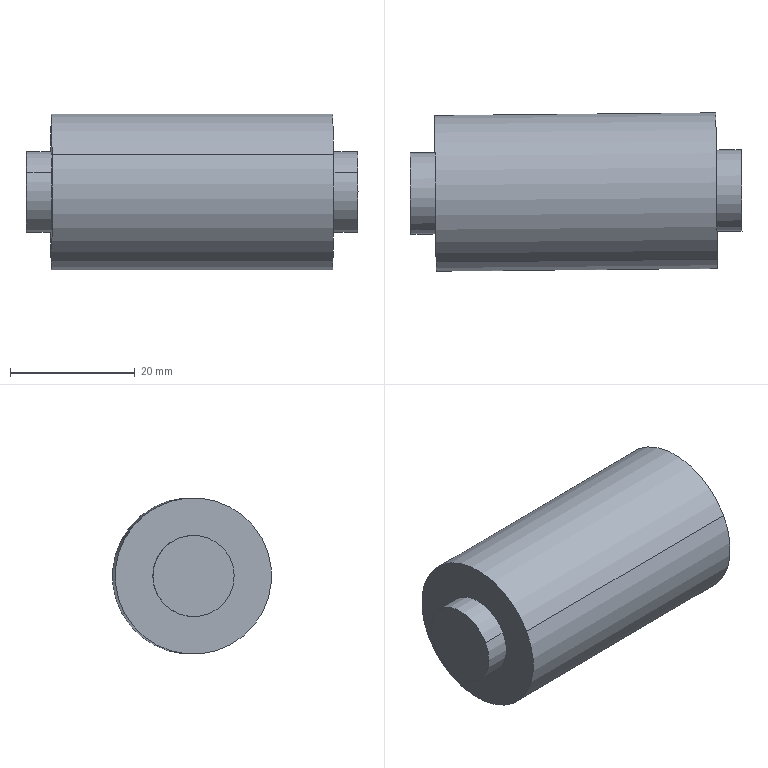Component | SolidWorks | CMAS50_F-2_CMAS50_Fbearing-1 | 1 solid | 10 faces | box 53.12 x 25.43 x 25 mm | volume 23151 mm3 | cylinder 6 | plane 4 | commonest cylinder face diameters 13 x4 25 x2 | material 45
build123d program:
from build123d import *


with BuildPart() as part:
    # Sketch1 → Revolve1 (revolve)
    with BuildSketch(Plane(origin=(0, 0, 0), x_dir=(0, 0, -1), z_dir=(1, 0, 0)), mode=Mode.PRIVATE) as revolve1_sk:
        Polygon((-26.5, 0), (-26.5, 6.5), (-22.5, 6.5), (-22.5, 12.5), (22.5, 12.5), (22.5, 6.5), (26.5, 6.5), (26.5, 0), align=None)
    revolve(revolve1_sk.sketch.rotate(Axis((0, 0, -26.5), (0, 0, 1)), 270), axis=Axis((0, 0, -26.5), (0, 0, 1)))


solid = part.part

# Placed as in the assembly
solid = solid.moved(Location((263.556, 604.998, 669), (-90, 89.448, -101.509)))
STEP:
#1=COLOUR_RGB('',0.7922,0.8196,0.9333);
#2=FILL_AREA_STYLE_COLOUR('',#1);
#3=FILL_AREA_STYLE('',(#2));
#4=SURFACE_STYLE_FILL_AREA(#3);
#5=SURFACE_SIDE_STYLE('',(#4));
#6=SURFACE_STYLE_USAGE(.BOTH.,#5);
#7=PRESENTATION_STYLE_ASSIGNMENT((#6));
#8=CARTESIAN_POINT('',(11.417,24.054,26.217));
#9=VERTEX_POINT('',#8);
#10=CARTESIAN_POINT('',(11.422,23.604,26.46));
#11=VERTEX_POINT('',#10);
#12=CARTESIAN_POINT('',(11.419,23.829,26.339));
#13=DIRECTION('',(-1.,-0.009642,0.));
#14=DIRECTION('',(-0.00848,0.8794,-0.476));
#15=AXIS2_PLACEMENT_3D('',#12,#13,#14);
#16=CIRCLE('',#15,0.2559);
#17=EDGE_CURVE('',#9,#11,#16,.T.);
#18=ORIENTED_EDGE('',*,*,#17,.T.);
#19=CARTESIAN_POINT('',(11.264,23.602,26.46));
#20=VERTEX_POINT('',#19);
#21=CARTESIAN_POINT('',(11.422,23.604,26.46));
#22=DIRECTION('',(-1.,-0.009642,0.));
#23=VECTOR('',#22,39.37);
#24=LINE('',#21,#23);
#25=EDGE_CURVE('',#11,#20,#24,.T.);
#26=ORIENTED_EDGE('',*,*,#25,.T.);
#27=CARTESIAN_POINT('',(11.26,24.052,26.217));
#28=VERTEX_POINT('',#27);
#29=CARTESIAN_POINT('',(11.262,23.827,26.339));
#30=DIRECTION('',(-1.,-0.009642,0.));
#31=DIRECTION('',(-0.00848,0.8794,-0.476));
#32=AXIS2_PLACEMENT_3D('',#29,#30,#31);
#33=CIRCLE('',#32,0.2559);
#34=EDGE_CURVE('',#28,#20,#33,.T.);
#35=ORIENTED_EDGE('',*,*,#34,.F.);
#36=CARTESIAN_POINT('',(11.417,24.054,26.217));
#37=DIRECTION('',(-1.,-0.009642,0.));
#38=VECTOR('',#37,39.37);
#39=LINE('',#36,#38);
#40=EDGE_CURVE('',#9,#28,#39,.T.);
#41=ORIENTED_EDGE('',*,*,#40,.F.);
#42=EDGE_LOOP('',(#18,#26,#35,#41));
#43=FACE_OUTER_BOUND('',#42,.T.);
#44=CARTESIAN_POINT('',(11.419,23.829,26.339));
#45=DIRECTION('',(-1.,-0.009642,0.));
#46=DIRECTION('',(-0.00848,0.8794,-0.476));
#47=AXIS2_PLACEMENT_3D('',#44,#45,#46);
#48=CYLINDRICAL_SURFACE('',#47,0.2559);
#49=ADVANCED_FACE('',(#43),#48,.T.);
#50=CARTESIAN_POINT('',(11.258,24.26,26.104));
#51=VERTEX_POINT('',#50);
#52=CARTESIAN_POINT('',(11.266,23.395,26.573));
#53=VERTEX_POINT('',#52);
#54=CARTESIAN_POINT('',(11.262,23.827,26.339));
#55=DIRECTION('',(-1.,-0.009642,0.));
#56=DIRECTION('',(-0.00848,0.8794,-0.476));
#57=AXIS2_PLACEMENT_3D('',#54,#55,#56);
#58=CIRCLE('',#57,0.4921);
#59=EDGE_CURVE('',#51,#53,#58,.T.);
#60=ORIENTED_EDGE('',*,*,#59,.T.);
#61=CARTESIAN_POINT('',(9.495,23.377,26.573));
#62=VERTEX_POINT('',#61);
#63=CARTESIAN_POINT('',(11.424,23.396,26.573));
#64=DIRECTION('',(-1.,-0.009642,0.));
#65=VECTOR('',#64,39.37);
#66=LINE('',#63,#65);
#67=EDGE_CURVE('',#53,#62,#66,.T.);
#68=ORIENTED_EDGE('',*,*,#67,.T.);
#69=CARTESIAN_POINT('',(9.486,24.243,26.104));
#70=VERTEX_POINT('',#69);
#71=CARTESIAN_POINT('',(9.49,23.81,26.339));
#72=DIRECTION('',(-1.,-0.009642,0.));
#73=DIRECTION('',(-0.00848,0.8794,-0.476));
#74=AXIS2_PLACEMENT_3D('',#71,#72,#73);
#75=CIRCLE('',#74,0.4921);
#76=EDGE_CURVE('',#70,#62,#75,.T.);
#77=ORIENTED_EDGE('',*,*,#76,.F.);
#78=CARTESIAN_POINT('',(11.415,24.262,26.104));
#79=DIRECTION('',(-1.,-0.009642,0.));
#80=VECTOR('',#79,39.37);
#81=LINE('',#78,#80);
#82=EDGE_CURVE('',#51,#70,#81,.T.);
#83=ORIENTED_EDGE('',*,*,#82,.F.);
#84=EDGE_LOOP('',(#60,#68,#77,#83));
#85=FACE_OUTER_BOUND('',#84,.T.);
#86=CARTESIAN_POINT('',(11.419,23.829,26.339));
#87=DIRECTION('',(-1.,-0.009642,0.));
#88=DIRECTION('',(-0.00848,0.8794,-0.476));
#89=AXIS2_PLACEMENT_3D('',#86,#87,#88);
#90=CYLINDRICAL_SURFACE('',#89,0.4921);
#91=ADVANCED_FACE('',(#85),#90,.T.);
#92=CARTESIAN_POINT('',(9.488,24.035,26.217));
#93=VERTEX_POINT('',#92);
#94=CARTESIAN_POINT('',(9.493,23.585,26.46));
#95=VERTEX_POINT('',#94);
#96=CARTESIAN_POINT('',(9.49,23.81,26.339));
#97=DIRECTION('',(-1.,-0.009642,0.));
#98=DIRECTION('',(-0.00848,0.8794,-0.476));
#99=AXIS2_PLACEMENT_3D('',#96,#97,#98);
#100=CIRCLE('',#99,0.2559);
#101=EDGE_CURVE('',#93,#95,#100,.T.);
#102=ORIENTED_EDGE('',*,*,#101,.T.);
#103=CARTESIAN_POINT('',(9.335,23.584,26.46));
#104=VERTEX_POINT('',#103);
#105=CARTESIAN_POINT('',(11.422,23.604,26.46));
#106=DIRECTION('',(-1.,-0.009642,0.));
#107=VECTOR('',#106,39.37);
#108=LINE('',#105,#107);
#109=EDGE_CURVE('',#95,#104,#108,.T.);
#110=ORIENTED_EDGE('',*,*,#109,.T.);
#111=CARTESIAN_POINT('',(9.331,24.034,26.217));
#112=VERTEX_POINT('',#111);
#113=CARTESIAN_POINT('',(9.333,23.809,26.339));
#114=DIRECTION('',(-1.,-0.009642,0.));
#115=DIRECTION('',(-0.00848,0.8794,-0.476));
#116=AXIS2_PLACEMENT_3D('',#113,#114,#115);
#117=CIRCLE('',#116,0.2559);
#118=EDGE_CURVE('',#112,#104,#117,.T.);
#119=ORIENTED_EDGE('',*,*,#118,.F.);
#120=CARTESIAN_POINT('',(11.417,24.054,26.217));
#121=DIRECTION('',(-1.,-0.009642,0.));
#122=VECTOR('',#121,39.37);
#123=LINE('',#120,#122);
#124=EDGE_CURVE('',#93,#112,#123,.T.);
#125=ORIENTED_EDGE('',*,*,#124,.F.);
#126=EDGE_LOOP('',(#102,#110,#119,#125));
#127=FACE_OUTER_BOUND('',#126,.T.);
#128=CARTESIAN_POINT('',(11.419,23.829,26.339));
#129=DIRECTION('',(-1.,-0.009642,0.));
#130=DIRECTION('',(-0.00848,0.8794,-0.476));
#131=AXIS2_PLACEMENT_3D('',#128,#129,#130);
#132=CYLINDRICAL_SURFACE('',#131,0.2559);
#133=ADVANCED_FACE('',(#127),#132,.T.);
#134=ORIENTED_EDGE('',*,*,#118,.T.);
#135=CARTESIAN_POINT('',(9.333,23.809,26.339));
#136=DIRECTION('',(-1.,-0.009642,0.));
#137=DIRECTION('',(-0.00848,0.8794,-0.476));
#138=AXIS2_PLACEMENT_3D('',#135,#136,#137);
#139=CIRCLE('',#138,0.2559);
#140=EDGE_CURVE('',#104,#112,#139,.T.);
#141=ORIENTED_EDGE('',*,*,#140,.T.);
#142=EDGE_LOOP('',(#134,#141));
#143=FACE_OUTER_BOUND('',#142,.T.);
#144=CARTESIAN_POINT('',(9.333,23.809,26.339));
#145=DIRECTION('',(1.,0.009642,-0.));
#146=DIRECTION('',(0.00848,-0.8794,0.476));
#147=AXIS2_PLACEMENT_3D('',#144,#145,#146);
#148=PLANE('',#147);
#149=ADVANCED_FACE('',(#143),#148,.F.);
#150=ORIENTED_EDGE('',*,*,#109,.F.);
#151=CARTESIAN_POINT('',(9.49,23.81,26.339));
#152=DIRECTION('',(-1.,-0.009642,0.));
#153=DIRECTION('',(-0.00848,0.8794,-0.476));
#154=AXIS2_PLACEMENT_3D('',#151,#152,#153);
#155=CIRCLE('',#154,0.2559);
#156=EDGE_CURVE('',#95,#93,#155,.T.);
#157=ORIENTED_EDGE('',*,*,#156,.T.);
#158=ORIENTED_EDGE('',*,*,#124,.T.);
#159=ORIENTED_EDGE('',*,*,#140,.F.);
#160=EDGE_LOOP('',(#150,#157,#158,#159));
#161=FACE_OUTER_BOUND('',#160,.T.);
#162=CARTESIAN_POINT('',(11.419,23.829,26.339));
#163=DIRECTION('',(-1.,-0.009642,0.));
#164=DIRECTION('',(-0.00848,0.8794,-0.476));
#165=AXIS2_PLACEMENT_3D('',#162,#163,#164);
#166=CYLINDRICAL_SURFACE('',#165,0.2559);
#167=ADVANCED_FACE('',(#161),#166,.T.);
#168=ORIENTED_EDGE('',*,*,#101,.F.);
#169=ORIENTED_EDGE('',*,*,#156,.F.);
#170=EDGE_LOOP('',(#168,#169));
#171=FACE_BOUND('',#170,.T.);
#172=ORIENTED_EDGE('',*,*,#76,.T.);
#173=CARTESIAN_POINT('',(9.49,23.81,26.339));
#174=DIRECTION('',(-1.,-0.009642,0.));
#175=DIRECTION('',(-0.00848,0.8794,-0.476));
#176=AXIS2_PLACEMENT_3D('',#173,#174,#175);
#177=CIRCLE('',#176,0.4921);
#178=EDGE_CURVE('',#62,#70,#177,.T.);
#179=ORIENTED_EDGE('',*,*,#178,.T.);
#180=EDGE_LOOP('',(#172,#179));
#181=FACE_OUTER_BOUND('',#180,.T.);
#182=CARTESIAN_POINT('',(9.492,23.688,26.114));
#183=DIRECTION('',(1.,0.009642,-0.));
#184=DIRECTION('',(0.00848,-0.8794,0.476));
#185=AXIS2_PLACEMENT_3D('',#182,#183,#184);
#186=PLANE('',#185);
#187=ADVANCED_FACE('',(#171,#181),#186,.F.);
#188=ORIENTED_EDGE('',*,*,#67,.F.);
#189=CARTESIAN_POINT('',(11.262,23.827,26.339));
#190=DIRECTION('',(-1.,-0.009642,0.));
#191=DIRECTION('',(-0.00848,0.8794,-0.476));
#192=AXIS2_PLACEMENT_3D('',#189,#190,#191);
#193=CIRCLE('',#192,0.4921);
#194=EDGE_CURVE('',#53,#51,#193,.T.);
#195=ORIENTED_EDGE('',*,*,#194,.T.);
#196=ORIENTED_EDGE('',*,*,#82,.T.);
#197=ORIENTED_EDGE('',*,*,#178,.F.);
#198=EDGE_LOOP('',(#188,#195,#196,#197));
#199=FACE_OUTER_BOUND('',#198,.T.);
#200=CARTESIAN_POINT('',(11.419,23.829,26.339));
#201=DIRECTION('',(-1.,-0.009642,0.));
#202=DIRECTION('',(-0.00848,0.8794,-0.476));
#203=AXIS2_PLACEMENT_3D('',#200,#201,#202);
#204=CYLINDRICAL_SURFACE('',#203,0.4921);
#205=ADVANCED_FACE('',(#199),#204,.T.);
#206=ORIENTED_EDGE('',*,*,#59,.F.);
#207=ORIENTED_EDGE('',*,*,#194,.F.);
#208=EDGE_LOOP('',(#206,#207));
#209=FACE_OUTER_BOUND('',#208,.T.);
#210=ORIENTED_EDGE('',*,*,#34,.T.);
#211=CARTESIAN_POINT('',(11.262,23.827,26.339));
#212=DIRECTION('',(-1.,-0.009642,0.));
#213=DIRECTION('',(-0.00848,0.8794,-0.476));
#214=AXIS2_PLACEMENT_3D('',#211,#212,#213);
#215=CIRCLE('',#214,0.2559);
#216=EDGE_CURVE('',#20,#28,#215,.T.);
#217=ORIENTED_EDGE('',*,*,#216,.T.);
#218=EDGE_LOOP('',(#210,#217));
#219=FACE_BOUND('',#218,.T.);
#220=CARTESIAN_POINT('',(11.264,23.593,25.906));
#221=DIRECTION('',(-1.,-0.009642,0.));
#222=DIRECTION('',(-0.00848,0.8794,-0.476));
#223=AXIS2_PLACEMENT_3D('',#220,#221,#222);
#224=PLANE('',#223);
#225=ADVANCED_FACE('',(#209,#219),#224,.F.);
#226=ORIENTED_EDGE('',*,*,#25,.F.);
#227=CARTESIAN_POINT('',(11.419,23.829,26.339));
#228=DIRECTION('',(-1.,-0.009642,0.));
#229=DIRECTION('',(-0.00848,0.8794,-0.476));
#230=AXIS2_PLACEMENT_3D('',#227,#228,#229);
#231=CIRCLE('',#230,0.2559);
#232=EDGE_CURVE('',#11,#9,#231,.T.);
#233=ORIENTED_EDGE('',*,*,#232,.T.);
#234=ORIENTED_EDGE('',*,*,#40,.T.);
#235=ORIENTED_EDGE('',*,*,#216,.F.);
#236=EDGE_LOOP('',(#226,#233,#234,#235));
#237=FACE_OUTER_BOUND('',#236,.T.);
#238=CARTESIAN_POINT('',(11.419,23.829,26.339));
#239=DIRECTION('',(-1.,-0.009642,0.));
#240=DIRECTION('',(-0.00848,0.8794,-0.476));
#241=AXIS2_PLACEMENT_3D('',#238,#239,#240);
#242=CYLINDRICAL_SURFACE('',#241,0.2559);
#243=ADVANCED_FACE('',(#237),#242,.T.);
#244=ORIENTED_EDGE('',*,*,#17,.F.);
#245=ORIENTED_EDGE('',*,*,#232,.F.);
#246=EDGE_LOOP('',(#244,#245));
#247=FACE_OUTER_BOUND('',#246,.T.);
#248=CARTESIAN_POINT('',(11.421,23.707,26.114));
#249=DIRECTION('',(-1.,-0.009642,0.));
#250=DIRECTION('',(-0.00848,0.8794,-0.476));
#251=AXIS2_PLACEMENT_3D('',#248,#249,#250);
#252=PLANE('',#251);
#253=ADVANCED_FACE('',(#247),#252,.F.);
#254=CLOSED_SHELL('',(#49,#91,#133,#149,#167,#187,#205,#225,#243,#253));
#255=MANIFOLD_SOLID_BREP('',#254);
#256=STYLED_ITEM('',(#7),#255);
#257=(LENGTH_UNIT()NAMED_UNIT(*)SI_UNIT($,.METRE.));
#258=LENGTH_MEASURE_WITH_UNIT(LENGTH_MEASURE(0.0254),#257);
#259=DIMENSIONAL_EXPONENTS(1.,0.,0.,0.,0.,0.,0.);
#260=(CONVERSION_BASED_UNIT('',#258)LENGTH_UNIT()NAMED_UNIT(#259));
#261=UNCERTAINTY_MEASURE_WITH_UNIT(LENGTH_MEASURE(0.00001),#260,'','');
#262=(NAMED_UNIT(*)PLANE_ANGLE_UNIT()SI_UNIT($,.RADIAN.));
#263=(NAMED_UNIT(*)SI_UNIT($,.STERADIAN.)SOLID_ANGLE_UNIT());
#264=(GEOMETRIC_REPRESENTATION_CONTEXT(3)GLOBAL_UNCERTAINTY_ASSIGNED_CONTEXT((#261))GLOBAL_UNIT_ASSIGNED_CONTEXT((#260,#262,#263))REPRESENTATION_CONTEXT('',''));
#265=MECHANICAL_DESIGN_GEOMETRIC_PRESENTATION_REPRESENTATION('',(#256),#264);
#266=PRESENTATION_LAYER_ASSIGNMENT('','',(#256));
#267=CARTESIAN_POINT('',(0.,0.,0.));
#268=DIRECTION('',(0.,0.,1.));
#269=DIRECTION('',(1.,0.,0.));
#270=AXIS2_PLACEMENT_3D('',#267,#268,#269);
#271=(LENGTH_UNIT()NAMED_UNIT(*)SI_UNIT($,.METRE.));
#272=LENGTH_MEASURE_WITH_UNIT(LENGTH_MEASURE(0.0254),#271);
#273=DIMENSIONAL_EXPONENTS(1.,0.,0.,0.,0.,0.,0.);
#274=(CONVERSION_BASED_UNIT('',#272)LENGTH_UNIT()NAMED_UNIT(#273));
#275=UNCERTAINTY_MEASURE_WITH_UNIT(LENGTH_MEASURE(0.00001),#274,'','');
#276=(NAMED_UNIT(*)PLANE_ANGLE_UNIT()SI_UNIT($,.RADIAN.));
#277=(NAMED_UNIT(*)SI_UNIT($,.STERADIAN.)SOLID_ANGLE_UNIT());
#278=(GEOMETRIC_REPRESENTATION_CONTEXT(3)GLOBAL_UNCERTAINTY_ASSIGNED_CONTEXT((#275))GLOBAL_UNIT_ASSIGNED_CONTEXT((#274,#276,#277))REPRESENTATION_CONTEXT('',''));
#279=ADVANCED_BREP_SHAPE_REPRESENTATION('',(#255,#270),#278);